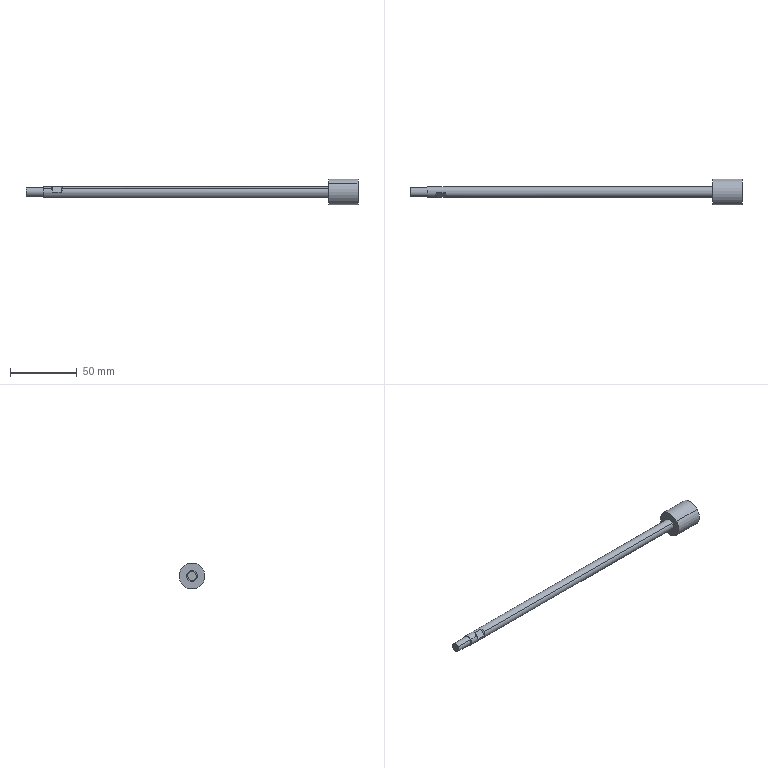Component | SolidWorks | CCDJSMA20x160SU(0)+(CS1-M-2)-1_CCDJS20UMA160 Rod-1 | 1 solid | 18 faces | box 249 x 19.5 x 19.5 mm | volume 17726 mm3 | plane 10 | cylinder 6 | cone 2 | commonest cylinder face diameters 6.647 x2 19.5 x2 8 x2
build123d program:
from build123d import *

# Parameters (mm, degrees)
CUT_EXTRUDE1_DEPTH      = 3
CUT_EXTRUDE1_DEPTH_BACK = 3
SKETCH1_W               = 13.5
SKETCH1_H               = 1.276


with BuildPart() as part:
    # Sketch1_2 → Revolve1 (revolve)
    with BuildSketch(Plane.XY, mode=Mode.PRIVATE) as revolve1_sk:
        Polygon((0, 0), (0, 3.233), (0.767, 4), (227, 4), (227, 9.75), (249, 9.75), (249, 0), align=None)
    revolve(revolve1_sk.sketch.rotate(Axis((249, 0, 0), (-1, 0, 0)), 270), axis=Axis((249, 0, 0), (-1, 0, 0)))

    # Sketch2 → Cut-Extrude1 (cut, two sides: drawn at the far end of the back side and taken through both)
    with BuildSketch(Plane(origin=(0, 0, 0), x_dir=(1, 0, 0), z_dir=(0, 1, 0)).offset(-CUT_EXTRUDE1_DEPTH_BACK)):
        Polygon((-5, -12), (35.4, -12), (26.4, -3), (20, -3), (18, -5), (18, -10), (-3, -10), (-3, 10), (18, 10), (18, 5), (20, 3), (26.4, 3), (35.4, 12), (-5, 12), align=None)
    extrude(amount=CUT_EXTRUDE1_DEPTH + CUT_EXTRUDE1_DEPTH_BACK, mode=Mode.SUBTRACT)

    # Sketch1 → Cut-Revolve1 (revolve, cut)
    with BuildSketch(Plane.XY, mode=Mode.PRIVATE) as cut_revolve1_sk:
        with Locations((6.25, 3.962)):
            Rectangle(SKETCH1_W, SKETCH1_H)
    revolve(cut_revolve1_sk.sketch.rotate(Axis((-1.5, 0, 0), (1, 0, 0)), 90), axis=Axis((-1.5, 0, 0), (1, 0, 0)), mode=Mode.SUBTRACT)


solid = part.part

# Placed as in the assembly
solid = solid.moved(Location((-92, 426.564, -63.57), (49.322, 0, 0)))
STEP:
#1=COLOUR_RGB('',0.7922,0.8196,0.9333);
#2=FILL_AREA_STYLE_COLOUR('',#1);
#3=FILL_AREA_STYLE('',(#2));
#4=SURFACE_STYLE_FILL_AREA(#3);
#5=SURFACE_SIDE_STYLE('',(#4));
#6=SURFACE_STYLE_USAGE(.BOTH.,#5);
#7=PRESENTATION_STYLE_ASSIGNMENT((#6));
#8=CARTESIAN_POINT('',(-3.622,16.89,-2.586));
#9=VERTEX_POINT('',#8);
#10=CARTESIAN_POINT('',(-3.622,16.697,-2.42));
#11=VERTEX_POINT('',#10);
#12=CARTESIAN_POINT('',(-3.622,16.794,-2.503));
#13=DIRECTION('',(-1.,0.,0.));
#14=DIRECTION('',(0.,0.7584,-0.6518));
#15=AXIS2_PLACEMENT_3D('',#12,#13,#14);
#16=CIRCLE('',#15,0.1273);
#17=EDGE_CURVE('',#9,#11,#16,.T.);
#18=ORIENTED_EDGE('',*,*,#17,.F.);
#19=CARTESIAN_POINT('',(-3.618,16.893,-2.588));
#20=VERTEX_POINT('',#19);
#21=CARTESIAN_POINT('',(-3.592,16.913,-2.605));
#22=DIRECTION('',(0.7071,0.5363,-0.4609));
#23=VECTOR('',#22,39.37);
#24=LINE('',#21,#23);
#25=EDGE_CURVE('',#9,#20,#24,.T.);
#26=ORIENTED_EDGE('',*,*,#25,.T.);
#27=CARTESIAN_POINT('',(-3.618,16.695,-2.417));
#28=VERTEX_POINT('',#27);
#29=CARTESIAN_POINT('',(-3.618,16.794,-2.503));
#30=DIRECTION('',(1.,0.,0.));
#31=DIRECTION('',(0.,-0.7584,0.6518));
#32=AXIS2_PLACEMENT_3D('',#29,#30,#31);
#33=CIRCLE('',#32,0.1308);
#34=EDGE_CURVE('',#28,#20,#33,.T.);
#35=ORIENTED_EDGE('',*,*,#34,.F.);
#36=CARTESIAN_POINT('',(-3.592,16.674,-2.4));
#37=DIRECTION('',(0.7071,-0.5363,0.4609));
#38=VECTOR('',#37,39.37);
#39=LINE('',#36,#38);
#40=EDGE_CURVE('',#11,#28,#39,.T.);
#41=ORIENTED_EDGE('',*,*,#40,.F.);
#42=EDGE_LOOP('',(#18,#26,#35,#41));
#43=FACE_OUTER_BOUND('',#42,.T.);
#44=CARTESIAN_POINT('',(-3.592,16.794,-2.503));
#45=DIRECTION('',(1.,0.,0.));
#46=DIRECTION('',(0.,-0.7584,0.6518));
#47=AXIS2_PLACEMENT_3D('',#44,#45,#46);
#48=CONICAL_SURFACE('',#47,0.1575,0.7854);
#49=ADVANCED_FACE('',(#43),#48,.T.);
#50=CARTESIAN_POINT('',(-3.11,16.893,-2.588));
#51=VERTEX_POINT('',#50);
#52=CARTESIAN_POINT('',(-3.11,16.695,-2.417));
#53=VERTEX_POINT('',#52);
#54=CARTESIAN_POINT('',(-3.11,16.794,-2.503));
#55=DIRECTION('',(-1.,0.,0.));
#56=DIRECTION('',(0.,0.7584,-0.6518));
#57=AXIS2_PLACEMENT_3D('',#54,#55,#56);
#58=CIRCLE('',#57,0.1308);
#59=EDGE_CURVE('',#51,#53,#58,.T.);
#60=ORIENTED_EDGE('',*,*,#59,.T.);
#61=CARTESIAN_POINT('',(-3.681,16.695,-2.417));
#62=DIRECTION('',(-1.,0.,0.));
#63=VECTOR('',#62,39.37);
#64=LINE('',#61,#63);
#65=EDGE_CURVE('',#53,#28,#64,.T.);
#66=ORIENTED_EDGE('',*,*,#65,.T.);
#67=ORIENTED_EDGE('',*,*,#34,.T.);
#68=CARTESIAN_POINT('',(-3.681,16.893,-2.588));
#69=DIRECTION('',(-1.,0.,0.));
#70=VECTOR('',#69,39.37);
#71=LINE('',#68,#70);
#72=EDGE_CURVE('',#51,#20,#71,.T.);
#73=ORIENTED_EDGE('',*,*,#72,.F.);
#74=EDGE_LOOP('',(#60,#66,#67,#73));
#75=FACE_OUTER_BOUND('',#74,.T.);
#76=CARTESIAN_POINT('',(-3.681,16.794,-2.503));
#77=DIRECTION('',(-1.,0.,0.));
#78=DIRECTION('',(0.,0.7584,-0.6518));
#79=AXIS2_PLACEMENT_3D('',#76,#77,#78);
#80=CYLINDRICAL_SURFACE('',#79,0.1308);
#81=ADVANCED_FACE('',(#75),#80,.T.);
#82=CARTESIAN_POINT('',(6.181,17.085,-2.753));
#83=VERTEX_POINT('',#82);
#84=CARTESIAN_POINT('',(6.181,16.503,-2.253));
#85=VERTEX_POINT('',#84);
#86=CARTESIAN_POINT('',(6.181,16.794,-2.503));
#87=DIRECTION('',(-1.,0.,0.));
#88=DIRECTION('',(0.,0.7584,-0.6518));
#89=AXIS2_PLACEMENT_3D('',#86,#87,#88);
#90=CIRCLE('',#89,0.3839);
#91=EDGE_CURVE('',#83,#85,#90,.T.);
#92=ORIENTED_EDGE('',*,*,#91,.T.);
#93=CARTESIAN_POINT('',(5.315,16.503,-2.253));
#94=VERTEX_POINT('',#93);
#95=CARTESIAN_POINT('',(6.181,16.503,-2.253));
#96=DIRECTION('',(-1.,0.,0.));
#97=VECTOR('',#96,39.37);
#98=LINE('',#95,#97);
#99=EDGE_CURVE('',#85,#94,#98,.T.);
#100=ORIENTED_EDGE('',*,*,#99,.T.);
#101=CARTESIAN_POINT('',(5.315,17.085,-2.753));
#102=VERTEX_POINT('',#101);
#103=CARTESIAN_POINT('',(5.315,16.794,-2.503));
#104=DIRECTION('',(-1.,0.,0.));
#105=DIRECTION('',(0.,0.7584,-0.6518));
#106=AXIS2_PLACEMENT_3D('',#103,#104,#105);
#107=CIRCLE('',#106,0.3839);
#108=EDGE_CURVE('',#102,#94,#107,.T.);
#109=ORIENTED_EDGE('',*,*,#108,.F.);
#110=CARTESIAN_POINT('',(6.181,17.085,-2.753));
#111=DIRECTION('',(-1.,0.,0.));
#112=VECTOR('',#111,39.37);
#113=LINE('',#110,#112);
#114=EDGE_CURVE('',#83,#102,#113,.T.);
#115=ORIENTED_EDGE('',*,*,#114,.F.);
#116=EDGE_LOOP('',(#92,#100,#109,#115));
#117=FACE_OUTER_BOUND('',#116,.T.);
#118=CARTESIAN_POINT('',(6.181,16.794,-2.503));
#119=DIRECTION('',(-1.,0.,0.));
#120=DIRECTION('',(0.,0.7584,-0.6518));
#121=AXIS2_PLACEMENT_3D('',#118,#119,#120);
#122=CYLINDRICAL_SURFACE('',#121,0.3839);
#123=ADVANCED_FACE('',(#117),#122,.T.);
#124=CARTESIAN_POINT('',(5.315,16.913,-2.605));
#125=VERTEX_POINT('',#124);
#126=CARTESIAN_POINT('',(5.315,16.674,-2.4));
#127=VERTEX_POINT('',#126);
#128=CARTESIAN_POINT('',(5.315,16.794,-2.503));
#129=DIRECTION('',(-1.,0.,0.));
#130=DIRECTION('',(0.,0.7584,-0.6518));
#131=AXIS2_PLACEMENT_3D('',#128,#129,#130);
#132=CIRCLE('',#131,0.1575);
#133=EDGE_CURVE('',#125,#127,#132,.T.);
#134=ORIENTED_EDGE('',*,*,#133,.T.);
#135=CARTESIAN_POINT('',(-2.543,16.674,-2.4));
#136=VERTEX_POINT('',#135);
#137=CARTESIAN_POINT('',(6.181,16.674,-2.4));
#138=DIRECTION('',(-1.,0.,0.));
#139=VECTOR('',#138,39.37);
#140=LINE('',#137,#139);
#141=EDGE_CURVE('',#127,#136,#140,.T.);
#142=ORIENTED_EDGE('',*,*,#141,.T.);
#143=CARTESIAN_POINT('',(-2.583,16.636,-2.505));
#144=VERTEX_POINT('',#143);
#145=CARTESIAN_POINT('',(-2.543,16.674,-2.4));
#146=CARTESIAN_POINT('',(-2.543,16.649,-2.43));
#147=CARTESIAN_POINT('',(-2.557,16.636,-2.466));
#148=CARTESIAN_POINT('',(-2.583,16.636,-2.505));
#149=(BOUNDED_CURVE()B_SPLINE_CURVE(3,(#145,#146,#147,#148),.UNSPECIFIED.,.F.,.F.)B_SPLINE_CURVE_WITH_KNOTS((4,4),(3.142,3.864),.UNSPECIFIED.)CURVE()GEOMETRIC_REPRESENTATION_ITEM()RATIONAL_B_SPLINE_CURVE((1.,0.9569,0.9569,1.))REPRESENTATION_ITEM(''));
#150=EDGE_CURVE('',#136,#144,#149,.T.);
#151=ORIENTED_EDGE('',*,*,#150,.T.);
#152=CARTESIAN_POINT('',(-2.835,16.636,-2.505));
#153=VERTEX_POINT('',#152);
#154=CARTESIAN_POINT('',(6.181,16.636,-2.505));
#155=DIRECTION('',(-1.,0.,0.));
#156=VECTOR('',#155,39.37);
#157=LINE('',#154,#156);
#158=EDGE_CURVE('',#144,#153,#157,.T.);
#159=ORIENTED_EDGE('',*,*,#158,.T.);
#160=CARTESIAN_POINT('',(-2.874,16.674,-2.4));
#161=VERTEX_POINT('',#160);
#162=CARTESIAN_POINT('',(-2.835,16.636,-2.505));
#163=CARTESIAN_POINT('',(-2.86,16.636,-2.466));
#164=CARTESIAN_POINT('',(-2.874,16.649,-2.43));
#165=CARTESIAN_POINT('',(-2.874,16.674,-2.4));
#166=(BOUNDED_CURVE()B_SPLINE_CURVE(3,(#162,#163,#164,#165),.UNSPECIFIED.,.F.,.F.)B_SPLINE_CURVE_WITH_KNOTS((4,4),(5.56,6.283),.UNSPECIFIED.)CURVE()GEOMETRIC_REPRESENTATION_ITEM()RATIONAL_B_SPLINE_CURVE((1.,0.9569,0.9569,1.))REPRESENTATION_ITEM(''));
#167=EDGE_CURVE('',#153,#161,#166,.T.);
#168=ORIENTED_EDGE('',*,*,#167,.T.);
#169=CARTESIAN_POINT('',(-3.11,16.674,-2.4));
#170=VERTEX_POINT('',#169);
#171=CARTESIAN_POINT('',(6.181,16.674,-2.4));
#172=DIRECTION('',(-1.,0.,0.));
#173=VECTOR('',#172,39.37);
#174=LINE('',#171,#173);
#175=EDGE_CURVE('',#161,#170,#174,.T.);
#176=ORIENTED_EDGE('',*,*,#175,.T.);
#177=CARTESIAN_POINT('',(-3.11,16.913,-2.605));
#178=VERTEX_POINT('',#177);
#179=CARTESIAN_POINT('',(-3.11,16.794,-2.503));
#180=DIRECTION('',(-1.,0.,0.));
#181=DIRECTION('',(0.,0.7584,-0.6518));
#182=AXIS2_PLACEMENT_3D('',#179,#180,#181);
#183=CIRCLE('',#182,0.1575);
#184=EDGE_CURVE('',#178,#170,#183,.T.);
#185=ORIENTED_EDGE('',*,*,#184,.F.);
#186=CARTESIAN_POINT('',(-2.874,16.913,-2.605));
#187=VERTEX_POINT('',#186);
#188=CARTESIAN_POINT('',(6.181,16.913,-2.605));
#189=DIRECTION('',(-1.,0.,0.));
#190=VECTOR('',#189,39.37);
#191=LINE('',#188,#190);
#192=EDGE_CURVE('',#187,#178,#191,.T.);
#193=ORIENTED_EDGE('',*,*,#192,.F.);
#194=CARTESIAN_POINT('',(-2.835,16.816,-2.659));
#195=VERTEX_POINT('',#194);
#196=CARTESIAN_POINT('',(-2.874,16.913,-2.605));
#197=CARTESIAN_POINT('',(-2.874,16.888,-2.635));
#198=CARTESIAN_POINT('',(-2.86,16.854,-2.653));
#199=CARTESIAN_POINT('',(-2.835,16.816,-2.659));
#200=(BOUNDED_CURVE()B_SPLINE_CURVE(3,(#196,#197,#198,#199),.UNSPECIFIED.,.F.,.F.)B_SPLINE_CURVE_WITH_KNOTS((4,4),(0.,0.7227),.UNSPECIFIED.)CURVE()GEOMETRIC_REPRESENTATION_ITEM()RATIONAL_B_SPLINE_CURVE((1.,0.9569,0.9569,1.))REPRESENTATION_ITEM(''));
#201=EDGE_CURVE('',#187,#195,#200,.T.);
#202=ORIENTED_EDGE('',*,*,#201,.T.);
#203=CARTESIAN_POINT('',(-2.583,16.816,-2.659));
#204=VERTEX_POINT('',#203);
#205=CARTESIAN_POINT('',(6.181,16.816,-2.659));
#206=DIRECTION('',(1.,0.,0.));
#207=VECTOR('',#206,39.37);
#208=LINE('',#205,#207);
#209=EDGE_CURVE('',#195,#204,#208,.T.);
#210=ORIENTED_EDGE('',*,*,#209,.T.);
#211=CARTESIAN_POINT('',(-2.543,16.913,-2.605));
#212=VERTEX_POINT('',#211);
#213=CARTESIAN_POINT('',(-2.583,16.816,-2.659));
#214=CARTESIAN_POINT('',(-2.557,16.854,-2.653));
#215=CARTESIAN_POINT('',(-2.543,16.888,-2.635));
#216=CARTESIAN_POINT('',(-2.543,16.913,-2.605));
#217=(BOUNDED_CURVE()B_SPLINE_CURVE(3,(#213,#214,#215,#216),.UNSPECIFIED.,.F.,.F.)B_SPLINE_CURVE_WITH_KNOTS((4,4),(2.419,3.142),.UNSPECIFIED.)CURVE()GEOMETRIC_REPRESENTATION_ITEM()RATIONAL_B_SPLINE_CURVE((1.,0.9569,0.9569,1.))REPRESENTATION_ITEM(''));
#218=EDGE_CURVE('',#204,#212,#217,.T.);
#219=ORIENTED_EDGE('',*,*,#218,.T.);
#220=CARTESIAN_POINT('',(6.181,16.913,-2.605));
#221=DIRECTION('',(-1.,0.,0.));
#222=VECTOR('',#221,39.37);
#223=LINE('',#220,#222);
#224=EDGE_CURVE('',#125,#212,#223,.T.);
#225=ORIENTED_EDGE('',*,*,#224,.F.);
#226=EDGE_LOOP('',(#134,#142,#151,#159,#168,#176,#185,#193,#202,#210,#219,#225));
#227=FACE_OUTER_BOUND('',#226,.T.);
#228=CARTESIAN_POINT('',(6.181,16.794,-2.503));
#229=DIRECTION('',(-1.,0.,0.));
#230=DIRECTION('',(0.,0.7584,-0.6518));
#231=AXIS2_PLACEMENT_3D('',#228,#229,#230);
#232=CYLINDRICAL_SURFACE('',#231,0.1575);
#233=ADVANCED_FACE('',(#227),#232,.T.);
#234=ORIENTED_EDGE('',*,*,#141,.F.);
#235=CARTESIAN_POINT('',(5.315,16.794,-2.503));
#236=DIRECTION('',(-1.,0.,0.));
#237=DIRECTION('',(0.,0.7584,-0.6518));
#238=AXIS2_PLACEMENT_3D('',#235,#236,#237);
#239=CIRCLE('',#238,0.1575);
#240=EDGE_CURVE('',#127,#125,#239,.T.);
#241=ORIENTED_EDGE('',*,*,#240,.T.);
#242=ORIENTED_EDGE('',*,*,#224,.T.);
#243=CARTESIAN_POINT('',(-2.583,16.951,-2.501));
#244=VERTEX_POINT('',#243);
#245=CARTESIAN_POINT('',(-2.543,16.913,-2.605));
#246=CARTESIAN_POINT('',(-2.543,16.939,-2.576));
#247=CARTESIAN_POINT('',(-2.557,16.952,-2.54));
#248=CARTESIAN_POINT('',(-2.583,16.951,-2.501));
#249=(BOUNDED_CURVE()B_SPLINE_CURVE(3,(#245,#246,#247,#248),.UNSPECIFIED.,.F.,.F.)B_SPLINE_CURVE_WITH_KNOTS((4,4),(3.142,3.864),.UNSPECIFIED.)CURVE()GEOMETRIC_REPRESENTATION_ITEM()RATIONAL_B_SPLINE_CURVE((1.,0.9569,0.9569,1.))REPRESENTATION_ITEM(''));
#250=EDGE_CURVE('',#212,#244,#249,.T.);
#251=ORIENTED_EDGE('',*,*,#250,.T.);
#252=CARTESIAN_POINT('',(-2.835,16.951,-2.501));
#253=VERTEX_POINT('',#252);
#254=CARTESIAN_POINT('',(6.181,16.951,-2.501));
#255=DIRECTION('',(-1.,0.,0.));
#256=VECTOR('',#255,39.37);
#257=LINE('',#254,#256);
#258=EDGE_CURVE('',#244,#253,#257,.T.);
#259=ORIENTED_EDGE('',*,*,#258,.T.);
#260=CARTESIAN_POINT('',(-2.835,16.951,-2.501));
#261=CARTESIAN_POINT('',(-2.86,16.952,-2.54));
#262=CARTESIAN_POINT('',(-2.874,16.939,-2.576));
#263=CARTESIAN_POINT('',(-2.874,16.913,-2.605));
#264=(BOUNDED_CURVE()B_SPLINE_CURVE(3,(#260,#261,#262,#263),.UNSPECIFIED.,.F.,.F.)B_SPLINE_CURVE_WITH_KNOTS((4,4),(5.56,6.283),.UNSPECIFIED.)CURVE()GEOMETRIC_REPRESENTATION_ITEM()RATIONAL_B_SPLINE_CURVE((1.,0.9569,0.9569,1.))REPRESENTATION_ITEM(''));
#265=EDGE_CURVE('',#253,#187,#264,.T.);
#266=ORIENTED_EDGE('',*,*,#265,.T.);
#267=ORIENTED_EDGE('',*,*,#192,.T.);
#268=CARTESIAN_POINT('',(-3.11,16.794,-2.503));
#269=DIRECTION('',(-1.,0.,0.));
#270=DIRECTION('',(0.,0.7584,-0.6518));
#271=AXIS2_PLACEMENT_3D('',#268,#269,#270);
#272=CIRCLE('',#271,0.1575);
#273=EDGE_CURVE('',#170,#178,#272,.T.);
#274=ORIENTED_EDGE('',*,*,#273,.F.);
#275=ORIENTED_EDGE('',*,*,#175,.F.);
#276=CARTESIAN_POINT('',(-2.835,16.772,-2.347));
#277=VERTEX_POINT('',#276);
#278=CARTESIAN_POINT('',(-2.874,16.674,-2.4));
#279=CARTESIAN_POINT('',(-2.874,16.7,-2.371));
#280=CARTESIAN_POINT('',(-2.86,16.734,-2.352));
#281=CARTESIAN_POINT('',(-2.835,16.772,-2.347));
#282=(BOUNDED_CURVE()B_SPLINE_CURVE(3,(#278,#279,#280,#281),.UNSPECIFIED.,.F.,.F.)B_SPLINE_CURVE_WITH_KNOTS((4,4),(0.,0.7227),.UNSPECIFIED.)CURVE()GEOMETRIC_REPRESENTATION_ITEM()RATIONAL_B_SPLINE_CURVE((1.,0.9569,0.9569,1.))REPRESENTATION_ITEM(''));
#283=EDGE_CURVE('',#161,#277,#282,.T.);
#284=ORIENTED_EDGE('',*,*,#283,.T.);
#285=CARTESIAN_POINT('',(-2.583,16.772,-2.347));
#286=VERTEX_POINT('',#285);
#287=CARTESIAN_POINT('',(6.181,16.772,-2.347));
#288=DIRECTION('',(1.,0.,0.));
#289=VECTOR('',#288,39.37);
#290=LINE('',#287,#289);
#291=EDGE_CURVE('',#277,#286,#290,.T.);
#292=ORIENTED_EDGE('',*,*,#291,.T.);
#293=CARTESIAN_POINT('',(-2.583,16.772,-2.347));
#294=CARTESIAN_POINT('',(-2.557,16.734,-2.352));
#295=CARTESIAN_POINT('',(-2.543,16.7,-2.371));
#296=CARTESIAN_POINT('',(-2.543,16.674,-2.4));
#297=(BOUNDED_CURVE()B_SPLINE_CURVE(3,(#293,#294,#295,#296),.UNSPECIFIED.,.F.,.F.)B_SPLINE_CURVE_WITH_KNOTS((4,4),(2.419,3.142),.UNSPECIFIED.)CURVE()GEOMETRIC_REPRESENTATION_ITEM()RATIONAL_B_SPLINE_CURVE((1.,0.9569,0.9569,1.))REPRESENTATION_ITEM(''));
#298=EDGE_CURVE('',#286,#136,#297,.T.);
#299=ORIENTED_EDGE('',*,*,#298,.T.);
#300=EDGE_LOOP('',(#234,#241,#242,#251,#259,#266,#267,#274,#275,#284,#292,#299));
#301=FACE_OUTER_BOUND('',#300,.T.);
#302=CARTESIAN_POINT('',(6.181,16.794,-2.503));
#303=DIRECTION('',(-1.,0.,0.));
#304=DIRECTION('',(0.,0.7584,-0.6518));
#305=AXIS2_PLACEMENT_3D('',#302,#303,#304);
#306=CYLINDRICAL_SURFACE('',#305,0.1575);
#307=ADVANCED_FACE('',(#301),#306,.T.);
#308=ORIENTED_EDGE('',*,*,#133,.F.);
#309=ORIENTED_EDGE('',*,*,#240,.F.);
#310=EDGE_LOOP('',(#308,#309));
#311=FACE_BOUND('',#310,.T.);
#312=ORIENTED_EDGE('',*,*,#108,.T.);
#313=CARTESIAN_POINT('',(5.315,16.794,-2.503));
#314=DIRECTION('',(-1.,0.,0.));
#315=DIRECTION('',(0.,0.7584,-0.6518));
#316=AXIS2_PLACEMENT_3D('',#313,#314,#315);
#317=CIRCLE('',#316,0.3839);
#318=EDGE_CURVE('',#94,#102,#317,.T.);
#319=ORIENTED_EDGE('',*,*,#318,.T.);
#320=EDGE_LOOP('',(#312,#319));
#321=FACE_OUTER_BOUND('',#320,.T.);
#322=CARTESIAN_POINT('',(5.315,16.691,-2.622));
#323=DIRECTION('',(1.,0.,0.));
#324=DIRECTION('',(0.,-0.7584,0.6518));
#325=AXIS2_PLACEMENT_3D('',#322,#323,#324);
#326=PLANE('',#325);
#327=ADVANCED_FACE('',(#311,#321),#326,.F.);
#328=ORIENTED_EDGE('',*,*,#99,.F.);
#329=CARTESIAN_POINT('',(6.181,16.794,-2.503));
#330=DIRECTION('',(-1.,0.,0.));
#331=DIRECTION('',(0.,0.7584,-0.6518));
#332=AXIS2_PLACEMENT_3D('',#329,#330,#331);
#333=CIRCLE('',#332,0.3839);
#334=EDGE_CURVE('',#85,#83,#333,.T.);
#335=ORIENTED_EDGE('',*,*,#334,.T.);
#336=ORIENTED_EDGE('',*,*,#114,.T.);
#337=ORIENTED_EDGE('',*,*,#318,.F.);
#338=EDGE_LOOP('',(#328,#335,#336,#337));
#339=FACE_OUTER_BOUND('',#338,.T.);
#340=CARTESIAN_POINT('',(6.181,16.794,-2.503));
#341=DIRECTION('',(-1.,0.,0.));
#342=DIRECTION('',(0.,0.7584,-0.6518));
#343=AXIS2_PLACEMENT_3D('',#340,#341,#342);
#344=CYLINDRICAL_SURFACE('',#343,0.3839);
#345=ADVANCED_FACE('',(#339),#344,.T.);
#346=ORIENTED_EDGE('',*,*,#91,.F.);
#347=ORIENTED_EDGE('',*,*,#334,.F.);
#348=EDGE_LOOP('',(#346,#347));
#349=FACE_OUTER_BOUND('',#348,.T.);
#350=CARTESIAN_POINT('',(6.181,16.544,-2.794));
#351=DIRECTION('',(-1.,0.,0.));
#352=DIRECTION('',(0.,0.7584,-0.6518));
#353=AXIS2_PLACEMENT_3D('',#350,#351,#352);
#354=PLANE('',#353);
#355=ADVANCED_FACE('',(#349),#354,.F.);
#356=CARTESIAN_POINT('',(-2.583,16.96,-2.49));
#357=DIRECTION('',(0.,-0.6518,-0.7584));
#358=VECTOR('',#357,39.37);
#359=LINE('',#356,#358);
#360=EDGE_CURVE('',#244,#204,#359,.T.);
#361=ORIENTED_EDGE('',*,*,#360,.F.);
#362=ORIENTED_EDGE('',*,*,#250,.F.);
#363=ORIENTED_EDGE('',*,*,#218,.F.);
#364=EDGE_LOOP('',(#361,#362,#363));
#365=FACE_OUTER_BOUND('',#364,.T.);
#366=CARTESIAN_POINT('',(-2.228,17.229,-2.721));
#367=DIRECTION('',(0.7071,-0.5363,0.4609));
#368=DIRECTION('',(-0.7071,-0.5363,0.4609));
#369=AXIS2_PLACEMENT_3D('',#366,#367,#368);
#370=PLANE('',#369);
#371=ADVANCED_FACE('',(#365),#370,.F.);
#372=ORIENTED_EDGE('',*,*,#360,.T.);
#373=ORIENTED_EDGE('',*,*,#209,.F.);
#374=CARTESIAN_POINT('',(-2.835,16.96,-2.49));
#375=DIRECTION('',(0.,-0.6518,-0.7584));
#376=VECTOR('',#375,39.37);
#377=LINE('',#374,#376);
#378=EDGE_CURVE('',#253,#195,#377,.T.);
#379=ORIENTED_EDGE('',*,*,#378,.F.);
#380=ORIENTED_EDGE('',*,*,#258,.F.);
#381=EDGE_LOOP('',(#372,#373,#379,#380));
#382=FACE_OUTER_BOUND('',#381,.T.);
#383=CARTESIAN_POINT('',(-2.583,16.96,-2.49));
#384=DIRECTION('',(0.,-0.7584,0.6518));
#385=DIRECTION('',(-1.,0.,0.));
#386=AXIS2_PLACEMENT_3D('',#383,#384,#385);
#387=PLANE('',#386);
#388=ADVANCED_FACE('',(#382),#387,.F.);
#389=ORIENTED_EDGE('',*,*,#378,.T.);
#390=ORIENTED_EDGE('',*,*,#201,.F.);
#391=ORIENTED_EDGE('',*,*,#265,.F.);
#392=EDGE_LOOP('',(#389,#390,#391));
#393=FACE_OUTER_BOUND('',#392,.T.);
#394=CARTESIAN_POINT('',(-2.835,16.96,-2.49));
#395=DIRECTION('',(-0.7071,-0.5363,0.4609));
#396=DIRECTION('',(-0.7071,0.5363,-0.4609));
#397=AXIS2_PLACEMENT_3D('',#394,#395,#396);
#398=PLANE('',#397);
#399=ADVANCED_FACE('',(#393),#398,.F.);
#400=CARTESIAN_POINT('',(-2.583,16.781,-2.336));
#401=DIRECTION('',(0.,-0.6518,-0.7584));
#402=VECTOR('',#401,39.37);
#403=LINE('',#400,#402);
#404=EDGE_CURVE('',#286,#144,#403,.T.);
#405=ORIENTED_EDGE('',*,*,#404,.T.);
#406=ORIENTED_EDGE('',*,*,#150,.F.);
#407=ORIENTED_EDGE('',*,*,#298,.F.);
#408=EDGE_LOOP('',(#405,#406,#407));
#409=FACE_OUTER_BOUND('',#408,.T.);
#410=CARTESIAN_POINT('',(-2.583,16.781,-2.336));
#411=DIRECTION('',(0.7071,0.5363,-0.4609));
#412=DIRECTION('',(0.7071,-0.5363,0.4609));
#413=AXIS2_PLACEMENT_3D('',#410,#411,#412);
#414=PLANE('',#413);
#415=ADVANCED_FACE('',(#409),#414,.F.);
#416=ORIENTED_EDGE('',*,*,#404,.F.);
#417=ORIENTED_EDGE('',*,*,#291,.F.);
#418=CARTESIAN_POINT('',(-2.835,16.781,-2.336));
#419=DIRECTION('',(0.,-0.6518,-0.7584));
#420=VECTOR('',#419,39.37);
#421=LINE('',#418,#420);
#422=EDGE_CURVE('',#277,#153,#421,.T.);
#423=ORIENTED_EDGE('',*,*,#422,.T.);
#424=ORIENTED_EDGE('',*,*,#158,.F.);
#425=EDGE_LOOP('',(#416,#417,#423,#424));
#426=FACE_OUTER_BOUND('',#425,.T.);
#427=CARTESIAN_POINT('',(-2.835,16.781,-2.336));
#428=DIRECTION('',(0.,0.7584,-0.6518));
#429=DIRECTION('',(1.,0.,0.));
#430=AXIS2_PLACEMENT_3D('',#427,#428,#429);
#431=PLANE('',#430);
#432=ADVANCED_FACE('',(#426),#431,.F.);
#433=ORIENTED_EDGE('',*,*,#422,.F.);
#434=ORIENTED_EDGE('',*,*,#283,.F.);
#435=ORIENTED_EDGE('',*,*,#167,.F.);
#436=EDGE_LOOP('',(#433,#434,#435));
#437=FACE_OUTER_BOUND('',#436,.T.);
#438=CARTESIAN_POINT('',(-2.913,16.722,-2.285));
#439=DIRECTION('',(-0.7071,0.5363,-0.4609));
#440=DIRECTION('',(0.7071,0.5363,-0.4609));
#441=AXIS2_PLACEMENT_3D('',#438,#439,#440);
#442=PLANE('',#441);
#443=ADVANCED_FACE('',(#437),#442,.F.);
#444=ORIENTED_EDGE('',*,*,#65,.F.);
#445=CARTESIAN_POINT('',(-3.11,16.794,-2.503));
#446=DIRECTION('',(-1.,0.,0.));
#447=DIRECTION('',(0.,0.7584,-0.6518));
#448=AXIS2_PLACEMENT_3D('',#445,#446,#447);
#449=CIRCLE('',#448,0.1308);
#450=EDGE_CURVE('',#53,#51,#449,.T.);
#451=ORIENTED_EDGE('',*,*,#450,.T.);
#452=ORIENTED_EDGE('',*,*,#72,.T.);
#453=CARTESIAN_POINT('',(-3.618,16.794,-2.503));
#454=DIRECTION('',(1.,0.,0.));
#455=DIRECTION('',(0.,-0.7584,0.6518));
#456=AXIS2_PLACEMENT_3D('',#453,#454,#455);
#457=CIRCLE('',#456,0.1308);
#458=EDGE_CURVE('',#20,#28,#457,.T.);
#459=ORIENTED_EDGE('',*,*,#458,.T.);
#460=EDGE_LOOP('',(#444,#451,#452,#459));
#461=FACE_OUTER_BOUND('',#460,.T.);
#462=CARTESIAN_POINT('',(-3.681,16.794,-2.503));
#463=DIRECTION('',(-1.,0.,0.));
#464=DIRECTION('',(0.,0.7584,-0.6518));
#465=AXIS2_PLACEMENT_3D('',#462,#463,#464);
#466=CYLINDRICAL_SURFACE('',#465,0.1308);
#467=ADVANCED_FACE('',(#461),#466,.T.);
#468=ORIENTED_EDGE('',*,*,#59,.F.);
#469=ORIENTED_EDGE('',*,*,#450,.F.);
#470=EDGE_LOOP('',(#468,#469));
#471=FACE_BOUND('',#470,.T.);
#472=ORIENTED_EDGE('',*,*,#184,.T.);
#473=ORIENTED_EDGE('',*,*,#273,.T.);
#474=EDGE_LOOP('',(#472,#473));
#475=FACE_OUTER_BOUND('',#474,.T.);
#476=CARTESIAN_POINT('',(-3.11,16.709,-2.602));
#477=DIRECTION('',(-1.,0.,0.));
#478=DIRECTION('',(0.,0.7584,-0.6518));
#479=AXIS2_PLACEMENT_3D('',#476,#477,#478);
#480=PLANE('',#479);
#481=ADVANCED_FACE('',(#471,#475),#480,.T.);
#482=CARTESIAN_POINT('',(-3.622,16.794,-2.503));
#483=DIRECTION('',(-1.,0.,0.));
#484=DIRECTION('',(0.,0.7584,-0.6518));
#485=AXIS2_PLACEMENT_3D('',#482,#483,#484);
#486=CIRCLE('',#485,0.1273);
#487=EDGE_CURVE('',#11,#9,#486,.T.);
#488=ORIENTED_EDGE('',*,*,#487,.T.);
#489=ORIENTED_EDGE('',*,*,#17,.T.);
#490=EDGE_LOOP('',(#488,#489));
#491=FACE_OUTER_BOUND('',#490,.T.);
#492=CARTESIAN_POINT('',(-3.622,16.794,-2.503));
#493=DIRECTION('',(1.,0.,0.));
#494=DIRECTION('',(0.,-0.7584,0.6518));
#495=AXIS2_PLACEMENT_3D('',#492,#493,#494);
#496=PLANE('',#495);
#497=ADVANCED_FACE('',(#491),#496,.F.);
#498=ORIENTED_EDGE('',*,*,#25,.F.);
#499=ORIENTED_EDGE('',*,*,#487,.F.);
#500=ORIENTED_EDGE('',*,*,#40,.T.);
#501=ORIENTED_EDGE('',*,*,#458,.F.);
#502=EDGE_LOOP('',(#498,#499,#500,#501));
#503=FACE_OUTER_BOUND('',#502,.T.);
#504=CARTESIAN_POINT('',(-3.592,16.794,-2.503));
#505=DIRECTION('',(1.,0.,0.));
#506=DIRECTION('',(0.,-0.7584,0.6518));
#507=AXIS2_PLACEMENT_3D('',#504,#505,#506);
#508=CONICAL_SURFACE('',#507,0.1575,0.7854);
#509=ADVANCED_FACE('',(#503),#508,.T.);
#510=CLOSED_SHELL('',(#49,#81,#123,#233,#307,#327,#345,#355,#371,#388,#399,#415,#432,#443,#467,#481,#497,#509));
#511=MANIFOLD_SOLID_BREP('',#510);
#512=STYLED_ITEM('',(#7),#511);
#513=PRESENTATION_LAYER_ASSIGNMENT('','',(#512));
#514=(LENGTH_UNIT()NAMED_UNIT(*)SI_UNIT($,.METRE.));
#515=LENGTH_MEASURE_WITH_UNIT(LENGTH_MEASURE(0.0254),#514);
#516=DIMENSIONAL_EXPONENTS(1.,0.,0.,0.,0.,0.,0.);
#517=(CONVERSION_BASED_UNIT('',#515)LENGTH_UNIT()NAMED_UNIT(#516));
#518=UNCERTAINTY_MEASURE_WITH_UNIT(LENGTH_MEASURE(0.00001),#517,'','');
#519=(NAMED_UNIT(*)PLANE_ANGLE_UNIT()SI_UNIT($,.RADIAN.));
#520=(NAMED_UNIT(*)SI_UNIT($,.STERADIAN.)SOLID_ANGLE_UNIT());
#521=(GEOMETRIC_REPRESENTATION_CONTEXT(3)GLOBAL_UNCERTAINTY_ASSIGNED_CONTEXT((#518))GLOBAL_UNIT_ASSIGNED_CONTEXT((#517,#519,#520))REPRESENTATION_CONTEXT('',''));
#522=MECHANICAL_DESIGN_GEOMETRIC_PRESENTATION_REPRESENTATION('',(#512),#521);
#523=CARTESIAN_POINT('',(0.,0.,0.));
#524=DIRECTION('',(0.,0.,1.));
#525=DIRECTION('',(1.,0.,0.));
#526=AXIS2_PLACEMENT_3D('',#523,#524,#525);
#527=(LENGTH_UNIT()NAMED_UNIT(*)SI_UNIT($,.METRE.));
#528=LENGTH_MEASURE_WITH_UNIT(LENGTH_MEASURE(0.0254),#527);
#529=DIMENSIONAL_EXPONENTS(1.,0.,0.,0.,0.,0.,0.);
#530=(CONVERSION_BASED_UNIT('',#528)LENGTH_UNIT()NAMED_UNIT(#529));
#531=UNCERTAINTY_MEASURE_WITH_UNIT(LENGTH_MEASURE(0.00001),#530,'','');
#532=(NAMED_UNIT(*)PLANE_ANGLE_UNIT()SI_UNIT($,.RADIAN.));
#533=(NAMED_UNIT(*)SI_UNIT($,.STERADIAN.)SOLID_ANGLE_UNIT());
#534=(GEOMETRIC_REPRESENTATION_CONTEXT(3)GLOBAL_UNCERTAINTY_ASSIGNED_CONTEXT((#531))GLOBAL_UNIT_ASSIGNED_CONTEXT((#530,#532,#533))REPRESENTATION_CONTEXT('',''));
#535=ADVANCED_BREP_SHAPE_REPRESENTATION('',(#511,#526),#534);